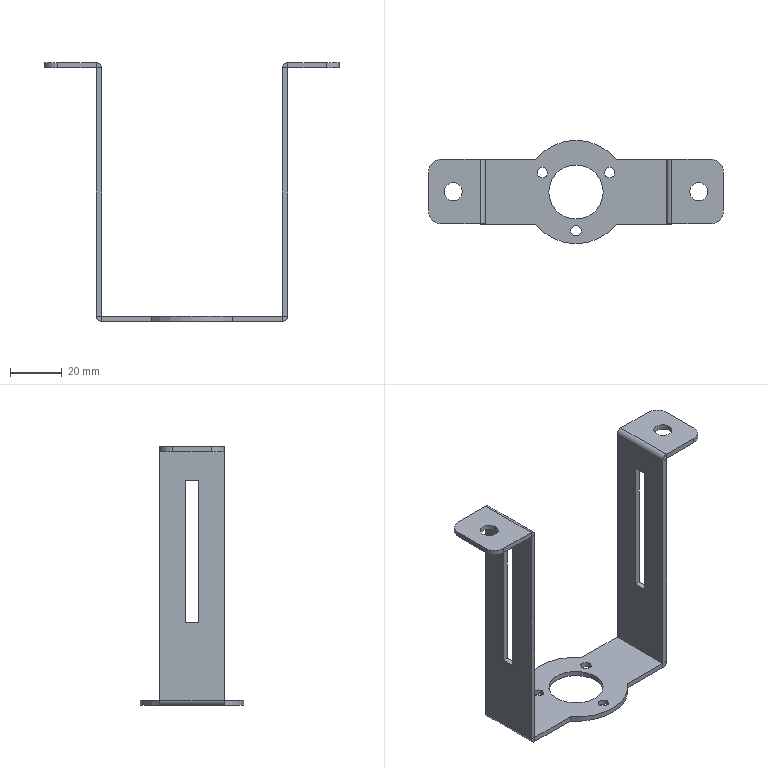Component | SolidWorks | 12AEncoderBracket-1 | 1 solid | 66 faces | volume 14002 mm3 | plane 40 | cylinder 26 | commonest cylinder face diameters 4 x6 7 x4 4.02 x4 0.02 x4 10 x4 21 x2 40 x2